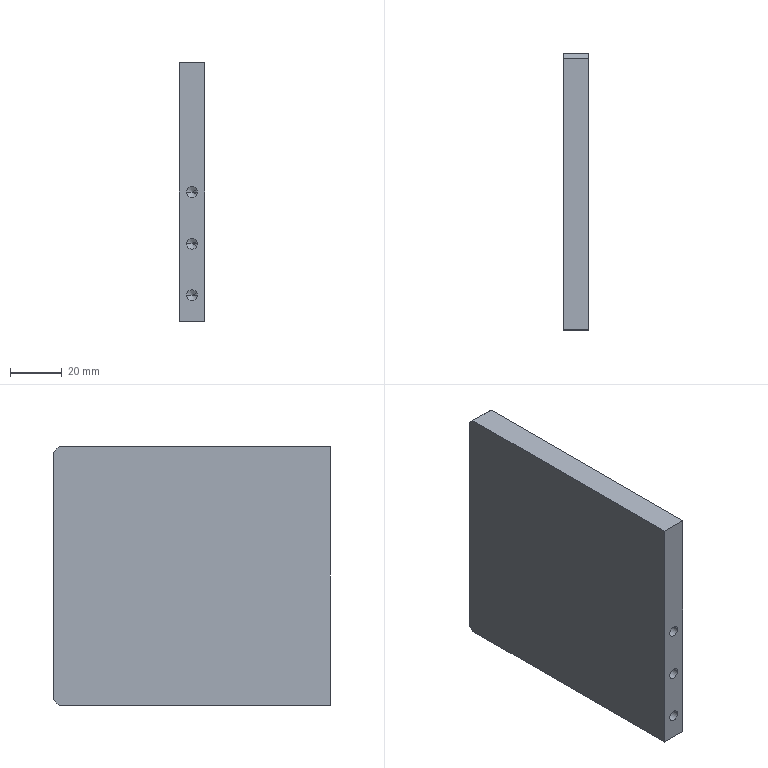Component | SolidWorks | AssemblyCylinderBracket54-1_SidePlate-2 | 1 solid | 20 faces | box 10 x 107 x 100 mm | volume 106361 mm3 | plane 8 | cylinder 6 | cone 6 | commonest cylinder face diameters 4.2 x6
build123d program:
from build123d import *

# Parameters (mm, degrees)
SKETCH1_W                 = 107
SKETCH1_H                 = 100
BOSS_EXTRUDE1_DEPTH       = 10
CHAMFER1_SIZE             = 2
M5X0_8_TAPPED_HOLE1_D     = 4.2
M5X0_8_TAPPED_HOLE1_DEPTH = 14
M5X0_8_TAPPED_HOLE1_TIP   = 1.262


with BuildPart() as part:
    # Sketch1 → Boss-Extrude1 (new body)
    with BuildSketch(Plane.XY):
        Rectangle(SKETCH1_W, SKETCH1_H)
    extrude(amount=BOSS_EXTRUDE1_DEPTH)

    # Chamfer1
    chamfer1_edges = [part.edges().sort_by_distance(p)[0] for p in [
        (-53.5, -50, 5),
        (-53.5, 50, 5),
    ]]
    chamfer(chamfer1_edges, length=CHAMFER1_SIZE)

    # M5x0.8 Tapped Hole1
    with Locations(Plane(origin=(53.5, 0, 0), x_dir=(0, 0, -1), z_dir=(1, 0, 0))):
        with Locations((-5, 40), (-5, 20), (-5, 0)):
            Hole(M5X0_8_TAPPED_HOLE1_D / 2, depth=M5X0_8_TAPPED_HOLE1_DEPTH)
            with Locations((0, 0, -(M5X0_8_TAPPED_HOLE1_DEPTH + M5X0_8_TAPPED_HOLE1_TIP / 2))):  # 118° drill point
                Cone(0, M5X0_8_TAPPED_HOLE1_D / 2, M5X0_8_TAPPED_HOLE1_TIP, mode=Mode.SUBTRACT)


solid = part.part

# Placed as in the assembly
solid = solid.moved(Location((135.085, -64.805, 51.359), (-90, 90, 0)))
STEP:
#1=CARTESIAN_POINT('',(5.598,-4.107,0.4472));
#2=VERTEX_POINT('',#1);
#3=CARTESIAN_POINT('',(5.432,-4.107,0.4472));
#4=VERTEX_POINT('',#3);
#5=CARTESIAN_POINT('',(5.515,-4.107,0.4472));
#6=DIRECTION('',(-0.,-1.,-0.));
#7=DIRECTION('',(-1.,0.,0.));
#8=AXIS2_PLACEMENT_3D('',#5,#6,#7);
#9=CIRCLE('',#8,0.08268);
#10=EDGE_CURVE('',#2,#4,#9,.T.);
#11=ORIENTED_EDGE('',*,*,#10,.F.);
#12=CARTESIAN_POINT('',(5.598,-4.658,0.4472));
#13=VERTEX_POINT('',#12);
#14=CARTESIAN_POINT('',(5.598,-4.658,0.4472));
#15=DIRECTION('',(-0.,-1.,-0.));
#16=VECTOR('',#15,39.37);
#17=LINE('',#14,#16);
#18=EDGE_CURVE('',#2,#13,#17,.T.);
#19=ORIENTED_EDGE('',*,*,#18,.T.);
#20=CARTESIAN_POINT('',(5.432,-4.658,0.4472));
#21=VERTEX_POINT('',#20);
#22=CARTESIAN_POINT('',(5.515,-4.658,0.4472));
#23=DIRECTION('',(-0.,-1.,-0.));
#24=DIRECTION('',(-1.,0.,0.));
#25=AXIS2_PLACEMENT_3D('',#22,#23,#24);
#26=CIRCLE('',#25,0.08268);
#27=EDGE_CURVE('',#13,#21,#26,.T.);
#28=ORIENTED_EDGE('',*,*,#27,.T.);
#29=CARTESIAN_POINT('',(5.432,-4.658,0.4472));
#30=DIRECTION('',(-0.,-1.,-0.));
#31=VECTOR('',#30,39.37);
#32=LINE('',#29,#31);
#33=EDGE_CURVE('',#4,#21,#32,.T.);
#34=ORIENTED_EDGE('',*,*,#33,.F.);
#35=EDGE_LOOP('',(#11,#19,#28,#34));
#36=FACE_OUTER_BOUND('',#35,.T.);
#37=CARTESIAN_POINT('',(5.515,-4.658,0.4472));
#38=DIRECTION('',(-0.,-1.,-0.));
#39=DIRECTION('',(-1.,0.,0.));
#40=AXIS2_PLACEMENT_3D('',#37,#38,#39);
#41=CYLINDRICAL_SURFACE('',#40,0.08268);
#42=ADVANCED_FACE('',(#36),#41,.F.);
#43=CARTESIAN_POINT('',(5.515,-4.057,0.4472));
#44=VERTEX_POINT('',#43);
#45=CARTESIAN_POINT('',(5.432,-4.107,0.4472));
#46=DIRECTION('',(-0.8572,-0.515,-0.));
#47=VECTOR('',#46,39.37);
#48=LINE('',#45,#47);
#49=EDGE_CURVE('',#44,#4,#48,.T.);
#50=ORIENTED_EDGE('',*,*,#49,.F.);
#51=CARTESIAN_POINT('',(5.598,-4.107,0.4472));
#52=DIRECTION('',(0.8572,-0.515,-0.));
#53=VECTOR('',#52,39.37);
#54=LINE('',#51,#53);
#55=EDGE_CURVE('',#44,#2,#54,.T.);
#56=ORIENTED_EDGE('',*,*,#55,.T.);
#57=ORIENTED_EDGE('',*,*,#10,.T.);
#58=EDGE_LOOP('',(#50,#56,#57));
#59=FACE_OUTER_BOUND('',#58,.T.);
#60=CARTESIAN_POINT('',(5.515,-4.107,0.4472));
#61=DIRECTION('',(-0.,-1.,-0.));
#62=DIRECTION('',(-1.,0.,0.));
#63=AXIS2_PLACEMENT_3D('',#60,#61,#62);
#64=CONICAL_SURFACE('',#63,0.08268,1.03);
#65=ADVANCED_FACE('',(#59),#64,.F.);
#66=CARTESIAN_POINT('',(5.598,-4.107,1.235));
#67=VERTEX_POINT('',#66);
#68=CARTESIAN_POINT('',(5.432,-4.107,1.235));
#69=VERTEX_POINT('',#68);
#70=CARTESIAN_POINT('',(5.515,-4.107,1.235));
#71=DIRECTION('',(-0.,-1.,-0.));
#72=DIRECTION('',(-1.,0.,0.));
#73=AXIS2_PLACEMENT_3D('',#70,#71,#72);
#74=CIRCLE('',#73,0.08268);
#75=EDGE_CURVE('',#67,#69,#74,.T.);
#76=ORIENTED_EDGE('',*,*,#75,.F.);
#77=CARTESIAN_POINT('',(5.598,-4.658,1.235));
#78=VERTEX_POINT('',#77);
#79=CARTESIAN_POINT('',(5.598,-4.658,1.235));
#80=DIRECTION('',(-0.,-1.,-0.));
#81=VECTOR('',#80,39.37);
#82=LINE('',#79,#81);
#83=EDGE_CURVE('',#67,#78,#82,.T.);
#84=ORIENTED_EDGE('',*,*,#83,.T.);
#85=CARTESIAN_POINT('',(5.432,-4.658,1.235));
#86=VERTEX_POINT('',#85);
#87=CARTESIAN_POINT('',(5.515,-4.658,1.235));
#88=DIRECTION('',(-0.,-1.,-0.));
#89=DIRECTION('',(-1.,0.,0.));
#90=AXIS2_PLACEMENT_3D('',#87,#88,#89);
#91=CIRCLE('',#90,0.08268);
#92=EDGE_CURVE('',#78,#86,#91,.T.);
#93=ORIENTED_EDGE('',*,*,#92,.T.);
#94=CARTESIAN_POINT('',(5.432,-4.658,1.235));
#95=DIRECTION('',(-0.,-1.,-0.));
#96=VECTOR('',#95,39.37);
#97=LINE('',#94,#96);
#98=EDGE_CURVE('',#69,#86,#97,.T.);
#99=ORIENTED_EDGE('',*,*,#98,.F.);
#100=EDGE_LOOP('',(#76,#84,#93,#99));
#101=FACE_OUTER_BOUND('',#100,.T.);
#102=CARTESIAN_POINT('',(5.515,-4.658,1.235));
#103=DIRECTION('',(-0.,-1.,-0.));
#104=DIRECTION('',(-1.,0.,0.));
#105=AXIS2_PLACEMENT_3D('',#102,#103,#104);
#106=CYLINDRICAL_SURFACE('',#105,0.08268);
#107=ADVANCED_FACE('',(#101),#106,.F.);
#108=CARTESIAN_POINT('',(5.515,-4.057,1.235));
#109=VERTEX_POINT('',#108);
#110=CARTESIAN_POINT('',(5.432,-4.107,1.235));
#111=DIRECTION('',(-0.8572,-0.515,-0.));
#112=VECTOR('',#111,39.37);
#113=LINE('',#110,#112);
#114=EDGE_CURVE('',#109,#69,#113,.T.);
#115=ORIENTED_EDGE('',*,*,#114,.F.);
#116=CARTESIAN_POINT('',(5.598,-4.107,1.235));
#117=DIRECTION('',(0.8572,-0.515,-0.));
#118=VECTOR('',#117,39.37);
#119=LINE('',#116,#118);
#120=EDGE_CURVE('',#109,#67,#119,.T.);
#121=ORIENTED_EDGE('',*,*,#120,.T.);
#122=ORIENTED_EDGE('',*,*,#75,.T.);
#123=EDGE_LOOP('',(#115,#121,#122));
#124=FACE_OUTER_BOUND('',#123,.T.);
#125=CARTESIAN_POINT('',(5.515,-4.107,1.235));
#126=DIRECTION('',(-0.,-1.,-0.));
#127=DIRECTION('',(-1.,0.,0.));
#128=AXIS2_PLACEMENT_3D('',#125,#126,#127);
#129=CONICAL_SURFACE('',#128,0.08268,1.03);
#130=ADVANCED_FACE('',(#124),#129,.F.);
#131=CARTESIAN_POINT('',(5.598,-4.107,2.022));
#132=VERTEX_POINT('',#131);
#133=CARTESIAN_POINT('',(5.432,-4.107,2.022));
#134=VERTEX_POINT('',#133);
#135=CARTESIAN_POINT('',(5.515,-4.107,2.022));
#136=DIRECTION('',(-0.,-1.,-0.));
#137=DIRECTION('',(-1.,0.,0.));
#138=AXIS2_PLACEMENT_3D('',#135,#136,#137);
#139=CIRCLE('',#138,0.08268);
#140=EDGE_CURVE('',#132,#134,#139,.T.);
#141=ORIENTED_EDGE('',*,*,#140,.F.);
#142=CARTESIAN_POINT('',(5.598,-4.658,2.022));
#143=VERTEX_POINT('',#142);
#144=CARTESIAN_POINT('',(5.598,-4.658,2.022));
#145=DIRECTION('',(-0.,-1.,-0.));
#146=VECTOR('',#145,39.37);
#147=LINE('',#144,#146);
#148=EDGE_CURVE('',#132,#143,#147,.T.);
#149=ORIENTED_EDGE('',*,*,#148,.T.);
#150=CARTESIAN_POINT('',(5.432,-4.658,2.022));
#151=VERTEX_POINT('',#150);
#152=CARTESIAN_POINT('',(5.515,-4.658,2.022));
#153=DIRECTION('',(-0.,-1.,-0.));
#154=DIRECTION('',(-1.,0.,0.));
#155=AXIS2_PLACEMENT_3D('',#152,#153,#154);
#156=CIRCLE('',#155,0.08268);
#157=EDGE_CURVE('',#143,#151,#156,.T.);
#158=ORIENTED_EDGE('',*,*,#157,.T.);
#159=CARTESIAN_POINT('',(5.432,-4.658,2.022));
#160=DIRECTION('',(-0.,-1.,-0.));
#161=VECTOR('',#160,39.37);
#162=LINE('',#159,#161);
#163=EDGE_CURVE('',#134,#151,#162,.T.);
#164=ORIENTED_EDGE('',*,*,#163,.F.);
#165=EDGE_LOOP('',(#141,#149,#158,#164));
#166=FACE_OUTER_BOUND('',#165,.T.);
#167=CARTESIAN_POINT('',(5.515,-4.658,2.022));
#168=DIRECTION('',(-0.,-1.,-0.));
#169=DIRECTION('',(-1.,0.,0.));
#170=AXIS2_PLACEMENT_3D('',#167,#168,#169);
#171=CYLINDRICAL_SURFACE('',#170,0.08268);
#172=ADVANCED_FACE('',(#166),#171,.F.);
#173=CARTESIAN_POINT('',(5.515,-4.057,2.022));
#174=VERTEX_POINT('',#173);
#175=CARTESIAN_POINT('',(5.432,-4.107,2.022));
#176=DIRECTION('',(-0.8572,-0.515,-0.));
#177=VECTOR('',#176,39.37);
#178=LINE('',#175,#177);
#179=EDGE_CURVE('',#174,#134,#178,.T.);
#180=ORIENTED_EDGE('',*,*,#179,.F.);
#181=CARTESIAN_POINT('',(5.598,-4.107,2.022));
#182=DIRECTION('',(0.8572,-0.515,-0.));
#183=VECTOR('',#182,39.37);
#184=LINE('',#181,#183);
#185=EDGE_CURVE('',#174,#132,#184,.T.);
#186=ORIENTED_EDGE('',*,*,#185,.T.);
#187=ORIENTED_EDGE('',*,*,#140,.T.);
#188=EDGE_LOOP('',(#180,#186,#187));
#189=FACE_OUTER_BOUND('',#188,.T.);
#190=CARTESIAN_POINT('',(5.515,-4.107,2.022));
#191=DIRECTION('',(-0.,-1.,-0.));
#192=DIRECTION('',(-1.,0.,0.));
#193=AXIS2_PLACEMENT_3D('',#190,#191,#192);
#194=CONICAL_SURFACE('',#193,0.08268,1.03);
#195=ADVANCED_FACE('',(#189),#194,.F.);
#196=CARTESIAN_POINT('',(5.515,-4.658,0.4472));
#197=DIRECTION('',(-0.,-1.,-0.));
#198=DIRECTION('',(-1.,0.,0.));
#199=AXIS2_PLACEMENT_3D('',#196,#197,#198);
#200=CIRCLE('',#199,0.08268);
#201=EDGE_CURVE('',#21,#13,#200,.T.);
#202=ORIENTED_EDGE('',*,*,#201,.F.);
#203=ORIENTED_EDGE('',*,*,#27,.F.);
#204=EDGE_LOOP('',(#202,#203));
#205=FACE_BOUND('',#204,.T.);
#206=CARTESIAN_POINT('',(5.515,-4.658,1.235));
#207=DIRECTION('',(-0.,-1.,-0.));
#208=DIRECTION('',(-1.,0.,0.));
#209=AXIS2_PLACEMENT_3D('',#206,#207,#208);
#210=CIRCLE('',#209,0.08268);
#211=EDGE_CURVE('',#86,#78,#210,.T.);
#212=ORIENTED_EDGE('',*,*,#211,.F.);
#213=ORIENTED_EDGE('',*,*,#92,.F.);
#214=EDGE_LOOP('',(#212,#213));
#215=FACE_BOUND('',#214,.T.);
#216=CARTESIAN_POINT('',(5.515,-4.658,2.022));
#217=DIRECTION('',(-0.,-1.,-0.));
#218=DIRECTION('',(-1.,0.,0.));
#219=AXIS2_PLACEMENT_3D('',#216,#217,#218);
#220=CIRCLE('',#219,0.08268);
#221=EDGE_CURVE('',#151,#143,#220,.T.);
#222=ORIENTED_EDGE('',*,*,#221,.F.);
#223=ORIENTED_EDGE('',*,*,#157,.F.);
#224=EDGE_LOOP('',(#222,#223));
#225=FACE_BOUND('',#224,.T.);
#226=CARTESIAN_POINT('',(5.318,-4.658,3.991));
#227=VERTEX_POINT('',#226);
#228=CARTESIAN_POINT('',(5.318,-4.658,0.0535));
#229=VERTEX_POINT('',#228);
#230=CARTESIAN_POINT('',(5.318,-4.658,0.0535));
#231=DIRECTION('',(0.,0.,-1.));
#232=VECTOR('',#231,39.37);
#233=LINE('',#230,#232);
#234=EDGE_CURVE('',#227,#229,#233,.T.);
#235=ORIENTED_EDGE('',*,*,#234,.T.);
#236=CARTESIAN_POINT('',(5.712,-4.658,0.0535));
#237=VERTEX_POINT('',#236);
#238=CARTESIAN_POINT('',(5.712,-4.658,0.0535));
#239=DIRECTION('',(-1.,0.,-0.));
#240=VECTOR('',#239,39.37);
#241=LINE('',#238,#240);
#242=EDGE_CURVE('',#237,#229,#241,.T.);
#243=ORIENTED_EDGE('',*,*,#242,.F.);
#244=CARTESIAN_POINT('',(5.712,-4.658,3.991));
#245=VERTEX_POINT('',#244);
#246=CARTESIAN_POINT('',(5.712,-4.658,0.0535));
#247=DIRECTION('',(0.,0.,-1.));
#248=VECTOR('',#247,39.37);
#249=LINE('',#246,#248);
#250=EDGE_CURVE('',#245,#237,#249,.T.);
#251=ORIENTED_EDGE('',*,*,#250,.F.);
#252=CARTESIAN_POINT('',(5.712,-4.658,3.991));
#253=DIRECTION('',(-1.,0.,-0.));
#254=VECTOR('',#253,39.37);
#255=LINE('',#252,#254);
#256=EDGE_CURVE('',#245,#227,#255,.T.);
#257=ORIENTED_EDGE('',*,*,#256,.T.);
#258=EDGE_LOOP('',(#235,#243,#251,#257));
#259=FACE_OUTER_BOUND('',#258,.T.);
#260=CARTESIAN_POINT('',(5.712,-4.658,0.0535));
#261=DIRECTION('',(0.,1.,0.));
#262=DIRECTION('',(-0.,-0.,1.));
#263=AXIS2_PLACEMENT_3D('',#260,#261,#262);
#264=PLANE('',#263);
#265=ADVANCED_FACE('',(#205,#215,#225,#259),#264,.F.);
#266=CARTESIAN_POINT('',(5.318,-0.5238,0.0535));
#267=VERTEX_POINT('',#266);
#268=CARTESIAN_POINT('',(5.318,-0.4451,0.0535));
#269=DIRECTION('',(0.,1.,0.));
#270=VECTOR('',#269,39.37);
#271=LINE('',#268,#270);
#272=EDGE_CURVE('',#229,#267,#271,.T.);
#273=ORIENTED_EDGE('',*,*,#272,.T.);
#274=CARTESIAN_POINT('',(5.712,-0.5238,0.0535));
#275=VERTEX_POINT('',#274);
#276=CARTESIAN_POINT('',(5.712,-0.5238,0.0535));
#277=DIRECTION('',(1.,-0.,0.));
#278=VECTOR('',#277,39.37);
#279=LINE('',#276,#278);
#280=EDGE_CURVE('',#267,#275,#279,.T.);
#281=ORIENTED_EDGE('',*,*,#280,.T.);
#282=CARTESIAN_POINT('',(5.712,-0.4451,0.0535));
#283=DIRECTION('',(0.,1.,0.));
#284=VECTOR('',#283,39.37);
#285=LINE('',#282,#284);
#286=EDGE_CURVE('',#237,#275,#285,.T.);
#287=ORIENTED_EDGE('',*,*,#286,.F.);
#288=ORIENTED_EDGE('',*,*,#242,.T.);
#289=EDGE_LOOP('',(#273,#281,#287,#288));
#290=FACE_OUTER_BOUND('',#289,.T.);
#291=CARTESIAN_POINT('',(5.712,-0.4451,0.0535));
#292=DIRECTION('',(-0.,-0.,1.));
#293=DIRECTION('',(-1.,0.,-0.));
#294=AXIS2_PLACEMENT_3D('',#291,#292,#293);
#295=PLANE('',#294);
#296=ADVANCED_FACE('',(#290),#295,.F.);
#297=CARTESIAN_POINT('',(5.318,-0.4451,0.1322));
#298=VERTEX_POINT('',#297);
#299=CARTESIAN_POINT('',(5.318,-0.4451,3.912));
#300=VERTEX_POINT('',#299);
#301=CARTESIAN_POINT('',(5.318,-0.4451,0.0535));
#302=DIRECTION('',(-0.,-0.,1.));
#303=VECTOR('',#302,39.37);
#304=LINE('',#301,#303);
#305=EDGE_CURVE('',#298,#300,#304,.T.);
#306=ORIENTED_EDGE('',*,*,#305,.T.);
#307=CARTESIAN_POINT('',(5.712,-0.4451,3.912));
#308=VERTEX_POINT('',#307);
#309=CARTESIAN_POINT('',(5.712,-0.4451,3.912));
#310=DIRECTION('',(1.,-0.,0.));
#311=VECTOR('',#310,39.37);
#312=LINE('',#309,#311);
#313=EDGE_CURVE('',#300,#308,#312,.T.);
#314=ORIENTED_EDGE('',*,*,#313,.T.);
#315=CARTESIAN_POINT('',(5.712,-0.4451,0.1322));
#316=VERTEX_POINT('',#315);
#317=CARTESIAN_POINT('',(5.712,-0.4451,0.0535));
#318=DIRECTION('',(-0.,-0.,1.));
#319=VECTOR('',#318,39.37);
#320=LINE('',#317,#319);
#321=EDGE_CURVE('',#316,#308,#320,.T.);
#322=ORIENTED_EDGE('',*,*,#321,.F.);
#323=CARTESIAN_POINT('',(5.712,-0.4451,0.1322));
#324=DIRECTION('',(-1.,0.,-0.));
#325=VECTOR('',#324,39.37);
#326=LINE('',#323,#325);
#327=EDGE_CURVE('',#316,#298,#326,.T.);
#328=ORIENTED_EDGE('',*,*,#327,.T.);
#329=EDGE_LOOP('',(#306,#314,#322,#328));
#330=FACE_OUTER_BOUND('',#329,.T.);
#331=CARTESIAN_POINT('',(5.712,-0.4451,0.0535));
#332=DIRECTION('',(-0.,-1.,-0.));
#333=DIRECTION('',(0.,0.,-1.));
#334=AXIS2_PLACEMENT_3D('',#331,#332,#333);
#335=PLANE('',#334);
#336=ADVANCED_FACE('',(#330),#335,.F.);
#337=CARTESIAN_POINT('',(5.712,-0.5238,3.991));
#338=VERTEX_POINT('',#337);
#339=CARTESIAN_POINT('',(5.712,-0.4451,3.991));
#340=DIRECTION('',(-0.,-1.,-0.));
#341=VECTOR('',#340,39.37);
#342=LINE('',#339,#341);
#343=EDGE_CURVE('',#338,#245,#342,.T.);
#344=ORIENTED_EDGE('',*,*,#343,.F.);
#345=CARTESIAN_POINT('',(5.318,-0.5238,3.991));
#346=VERTEX_POINT('',#345);
#347=CARTESIAN_POINT('',(5.712,-0.5238,3.991));
#348=DIRECTION('',(-1.,0.,-0.));
#349=VECTOR('',#348,39.37);
#350=LINE('',#347,#349);
#351=EDGE_CURVE('',#338,#346,#350,.T.);
#352=ORIENTED_EDGE('',*,*,#351,.T.);
#353=CARTESIAN_POINT('',(5.318,-0.4451,3.991));
#354=DIRECTION('',(-0.,-1.,-0.));
#355=VECTOR('',#354,39.37);
#356=LINE('',#353,#355);
#357=EDGE_CURVE('',#346,#227,#356,.T.);
#358=ORIENTED_EDGE('',*,*,#357,.T.);
#359=ORIENTED_EDGE('',*,*,#256,.F.);
#360=EDGE_LOOP('',(#344,#352,#358,#359));
#361=FACE_OUTER_BOUND('',#360,.T.);
#362=CARTESIAN_POINT('',(5.712,-0.4451,3.991));
#363=DIRECTION('',(0.,0.,-1.));
#364=DIRECTION('',(1.,-0.,0.));
#365=AXIS2_PLACEMENT_3D('',#362,#363,#364);
#366=PLANE('',#365);
#367=ADVANCED_FACE('',(#361),#366,.F.);
#368=ORIENTED_EDGE('',*,*,#321,.T.);
#369=CARTESIAN_POINT('',(5.712,-0.5534,4.02));
#370=DIRECTION('',(-0.,-0.7071,0.7071));
#371=VECTOR('',#370,39.37);
#372=LINE('',#369,#371);
#373=EDGE_CURVE('',#308,#338,#372,.T.);
#374=ORIENTED_EDGE('',*,*,#373,.T.);
#375=ORIENTED_EDGE('',*,*,#343,.T.);
#376=ORIENTED_EDGE('',*,*,#250,.T.);
#377=ORIENTED_EDGE('',*,*,#286,.T.);
#378=CARTESIAN_POINT('',(5.712,-0.5534,0.02398));
#379=DIRECTION('',(0.,0.7071,0.7071));
#380=VECTOR('',#379,39.37);
#381=LINE('',#378,#380);
#382=EDGE_CURVE('',#275,#316,#381,.T.);
#383=ORIENTED_EDGE('',*,*,#382,.T.);
#384=EDGE_LOOP('',(#368,#374,#375,#376,#377,#383));
#385=FACE_OUTER_BOUND('',#384,.T.);
#386=CARTESIAN_POINT('',(5.712,-2.551,2.022));
#387=DIRECTION('',(1.,-0.,0.));
#388=DIRECTION('',(-0.,-1.,-0.));
#389=AXIS2_PLACEMENT_3D('',#386,#387,#388);
#390=PLANE('',#389);
#391=ADVANCED_FACE('',(#385),#390,.T.);
#392=ORIENTED_EDGE('',*,*,#357,.F.);
#393=CARTESIAN_POINT('',(5.318,-0.5238,3.991));
#394=DIRECTION('',(0.,0.7071,-0.7071));
#395=VECTOR('',#394,39.37);
#396=LINE('',#393,#395);
#397=EDGE_CURVE('',#346,#300,#396,.T.);
#398=ORIENTED_EDGE('',*,*,#397,.T.);
#399=ORIENTED_EDGE('',*,*,#305,.F.);
#400=CARTESIAN_POINT('',(5.318,-0.4451,0.1322));
#401=DIRECTION('',(-0.,-0.7071,-0.7071));
#402=VECTOR('',#401,39.37);
#403=LINE('',#400,#402);
#404=EDGE_CURVE('',#298,#267,#403,.T.);
#405=ORIENTED_EDGE('',*,*,#404,.T.);
#406=ORIENTED_EDGE('',*,*,#272,.F.);
#407=ORIENTED_EDGE('',*,*,#234,.F.);
#408=EDGE_LOOP('',(#392,#398,#399,#405,#406,#407));
#409=FACE_OUTER_BOUND('',#408,.T.);
#410=CARTESIAN_POINT('',(5.318,-2.551,2.022));
#411=DIRECTION('',(1.,-0.,0.));
#412=DIRECTION('',(-0.,-1.,-0.));
#413=AXIS2_PLACEMENT_3D('',#410,#411,#412);
#414=PLANE('',#413);
#415=ADVANCED_FACE('',(#409),#414,.F.);
#416=ORIENTED_EDGE('',*,*,#373,.F.);
#417=ORIENTED_EDGE('',*,*,#313,.F.);
#418=ORIENTED_EDGE('',*,*,#397,.F.);
#419=ORIENTED_EDGE('',*,*,#351,.F.);
#420=EDGE_LOOP('',(#416,#417,#418,#419));
#421=FACE_OUTER_BOUND('',#420,.T.);
#422=CARTESIAN_POINT('',(5.712,-0.5238,3.991));
#423=DIRECTION('',(-0.,-0.7071,-0.7071));
#424=DIRECTION('',(-1.,0.,-0.));
#425=AXIS2_PLACEMENT_3D('',#422,#423,#424);
#426=PLANE('',#425);
#427=ADVANCED_FACE('',(#421),#426,.F.);
#428=ORIENTED_EDGE('',*,*,#382,.F.);
#429=ORIENTED_EDGE('',*,*,#280,.F.);
#430=ORIENTED_EDGE('',*,*,#404,.F.);
#431=ORIENTED_EDGE('',*,*,#327,.F.);
#432=EDGE_LOOP('',(#428,#429,#430,#431));
#433=FACE_OUTER_BOUND('',#432,.T.);
#434=CARTESIAN_POINT('',(5.712,-0.4451,0.1322));
#435=DIRECTION('',(-0.,-0.7071,0.7071));
#436=DIRECTION('',(-1.,0.,-0.));
#437=AXIS2_PLACEMENT_3D('',#434,#435,#436);
#438=PLANE('',#437);
#439=ADVANCED_FACE('',(#433),#438,.F.);
#440=ORIENTED_EDGE('',*,*,#185,.F.);
#441=ORIENTED_EDGE('',*,*,#179,.T.);
#442=CARTESIAN_POINT('',(5.515,-4.107,2.022));
#443=DIRECTION('',(-0.,-1.,-0.));
#444=DIRECTION('',(-1.,0.,0.));
#445=AXIS2_PLACEMENT_3D('',#442,#443,#444);
#446=CIRCLE('',#445,0.08268);
#447=EDGE_CURVE('',#134,#132,#446,.T.);
#448=ORIENTED_EDGE('',*,*,#447,.T.);
#449=EDGE_LOOP('',(#440,#441,#448));
#450=FACE_OUTER_BOUND('',#449,.T.);
#451=CARTESIAN_POINT('',(5.515,-4.107,2.022));
#452=DIRECTION('',(-0.,-1.,-0.));
#453=DIRECTION('',(-1.,0.,0.));
#454=AXIS2_PLACEMENT_3D('',#451,#452,#453);
#455=CONICAL_SURFACE('',#454,0.08268,1.03);
#456=ADVANCED_FACE('',(#450),#455,.F.);
#457=ORIENTED_EDGE('',*,*,#148,.F.);
#458=ORIENTED_EDGE('',*,*,#447,.F.);
#459=ORIENTED_EDGE('',*,*,#163,.T.);
#460=ORIENTED_EDGE('',*,*,#221,.T.);
#461=EDGE_LOOP('',(#457,#458,#459,#460));
#462=FACE_OUTER_BOUND('',#461,.T.);
#463=CARTESIAN_POINT('',(5.515,-4.658,2.022));
#464=DIRECTION('',(-0.,-1.,-0.));
#465=DIRECTION('',(-1.,0.,0.));
#466=AXIS2_PLACEMENT_3D('',#463,#464,#465);
#467=CYLINDRICAL_SURFACE('',#466,0.08268);
#468=ADVANCED_FACE('',(#462),#467,.F.);
#469=ORIENTED_EDGE('',*,*,#120,.F.);
#470=ORIENTED_EDGE('',*,*,#114,.T.);
#471=CARTESIAN_POINT('',(5.515,-4.107,1.235));
#472=DIRECTION('',(-0.,-1.,-0.));
#473=DIRECTION('',(-1.,0.,0.));
#474=AXIS2_PLACEMENT_3D('',#471,#472,#473);
#475=CIRCLE('',#474,0.08268);
#476=EDGE_CURVE('',#69,#67,#475,.T.);
#477=ORIENTED_EDGE('',*,*,#476,.T.);
#478=EDGE_LOOP('',(#469,#470,#477));
#479=FACE_OUTER_BOUND('',#478,.T.);
#480=CARTESIAN_POINT('',(5.515,-4.107,1.235));
#481=DIRECTION('',(-0.,-1.,-0.));
#482=DIRECTION('',(-1.,0.,0.));
#483=AXIS2_PLACEMENT_3D('',#480,#481,#482);
#484=CONICAL_SURFACE('',#483,0.08268,1.03);
#485=ADVANCED_FACE('',(#479),#484,.F.);
#486=ORIENTED_EDGE('',*,*,#83,.F.);
#487=ORIENTED_EDGE('',*,*,#476,.F.);
#488=ORIENTED_EDGE('',*,*,#98,.T.);
#489=ORIENTED_EDGE('',*,*,#211,.T.);
#490=EDGE_LOOP('',(#486,#487,#488,#489));
#491=FACE_OUTER_BOUND('',#490,.T.);
#492=CARTESIAN_POINT('',(5.515,-4.658,1.235));
#493=DIRECTION('',(-0.,-1.,-0.));
#494=DIRECTION('',(-1.,0.,0.));
#495=AXIS2_PLACEMENT_3D('',#492,#493,#494);
#496=CYLINDRICAL_SURFACE('',#495,0.08268);
#497=ADVANCED_FACE('',(#491),#496,.F.);
#498=ORIENTED_EDGE('',*,*,#55,.F.);
#499=ORIENTED_EDGE('',*,*,#49,.T.);
#500=CARTESIAN_POINT('',(5.515,-4.107,0.4472));
#501=DIRECTION('',(-0.,-1.,-0.));
#502=DIRECTION('',(-1.,0.,0.));
#503=AXIS2_PLACEMENT_3D('',#500,#501,#502);
#504=CIRCLE('',#503,0.08268);
#505=EDGE_CURVE('',#4,#2,#504,.T.);
#506=ORIENTED_EDGE('',*,*,#505,.T.);
#507=EDGE_LOOP('',(#498,#499,#506));
#508=FACE_OUTER_BOUND('',#507,.T.);
#509=CARTESIAN_POINT('',(5.515,-4.107,0.4472));
#510=DIRECTION('',(-0.,-1.,-0.));
#511=DIRECTION('',(-1.,0.,0.));
#512=AXIS2_PLACEMENT_3D('',#509,#510,#511);
#513=CONICAL_SURFACE('',#512,0.08268,1.03);
#514=ADVANCED_FACE('',(#508),#513,.F.);
#515=ORIENTED_EDGE('',*,*,#18,.F.);
#516=ORIENTED_EDGE('',*,*,#505,.F.);
#517=ORIENTED_EDGE('',*,*,#33,.T.);
#518=ORIENTED_EDGE('',*,*,#201,.T.);
#519=EDGE_LOOP('',(#515,#516,#517,#518));
#520=FACE_OUTER_BOUND('',#519,.T.);
#521=CARTESIAN_POINT('',(5.515,-4.658,0.4472));
#522=DIRECTION('',(-0.,-1.,-0.));
#523=DIRECTION('',(-1.,0.,0.));
#524=AXIS2_PLACEMENT_3D('',#521,#522,#523);
#525=CYLINDRICAL_SURFACE('',#524,0.08268);
#526=ADVANCED_FACE('',(#520),#525,.F.);
#527=CLOSED_SHELL('',(#42,#65,#107,#130,#172,#195,#265,#296,#336,#367,#391,#415,#427,#439,#456,#468,#485,#497,#514,#526));
#528=MANIFOLD_SOLID_BREP('',#527);
#529=CARTESIAN_POINT('',(0.,0.,0.));
#530=DIRECTION('',(0.,0.,1.));
#531=DIRECTION('',(1.,0.,0.));
#532=AXIS2_PLACEMENT_3D('',#529,#530,#531);
#533=(LENGTH_UNIT()NAMED_UNIT(*)SI_UNIT($,.METRE.));
#534=LENGTH_MEASURE_WITH_UNIT(LENGTH_MEASURE(0.0254),#533);
#535=DIMENSIONAL_EXPONENTS(1.,0.,0.,0.,0.,0.,0.);
#536=(CONVERSION_BASED_UNIT('',#534)LENGTH_UNIT()NAMED_UNIT(#535));
#537=UNCERTAINTY_MEASURE_WITH_UNIT(LENGTH_MEASURE(0.00001),#536,'','');
#538=(NAMED_UNIT(*)PLANE_ANGLE_UNIT()SI_UNIT($,.RADIAN.));
#539=(NAMED_UNIT(*)SI_UNIT($,.STERADIAN.)SOLID_ANGLE_UNIT());
#540=(GEOMETRIC_REPRESENTATION_CONTEXT(3)GLOBAL_UNCERTAINTY_ASSIGNED_CONTEXT((#537))GLOBAL_UNIT_ASSIGNED_CONTEXT((#536,#538,#539))REPRESENTATION_CONTEXT('',''));
#541=ADVANCED_BREP_SHAPE_REPRESENTATION('',(#528,#532),#540);
#542=COLOUR_RGB('',0.7922,0.8196,0.9333);
#543=FILL_AREA_STYLE_COLOUR('',#542);
#544=FILL_AREA_STYLE('',(#543));
#545=SURFACE_STYLE_FILL_AREA(#544);
#546=SURFACE_SIDE_STYLE('',(#545));
#547=SURFACE_STYLE_USAGE(.BOTH.,#546);
#548=PRESENTATION_STYLE_ASSIGNMENT((#547));
#549=STYLED_ITEM('',(#548),#528);
#550=(LENGTH_UNIT()NAMED_UNIT(*)SI_UNIT($,.METRE.));
#551=LENGTH_MEASURE_WITH_UNIT(LENGTH_MEASURE(0.0254),#550);
#552=DIMENSIONAL_EXPONENTS(1.,0.,0.,0.,0.,0.,0.);
#553=(CONVERSION_BASED_UNIT('',#551)LENGTH_UNIT()NAMED_UNIT(#552));
#554=UNCERTAINTY_MEASURE_WITH_UNIT(LENGTH_MEASURE(0.00001),#553,'','');
#555=(NAMED_UNIT(*)PLANE_ANGLE_UNIT()SI_UNIT($,.RADIAN.));
#556=(NAMED_UNIT(*)SI_UNIT($,.STERADIAN.)SOLID_ANGLE_UNIT());
#557=(GEOMETRIC_REPRESENTATION_CONTEXT(3)GLOBAL_UNCERTAINTY_ASSIGNED_CONTEXT((#554))GLOBAL_UNIT_ASSIGNED_CONTEXT((#553,#555,#556))REPRESENTATION_CONTEXT('',''));
#558=MECHANICAL_DESIGN_GEOMETRIC_PRESENTATION_REPRESENTATION('',(#549),#557);
#559=PRESENTATION_LAYER_ASSIGNMENT('','',(#549));